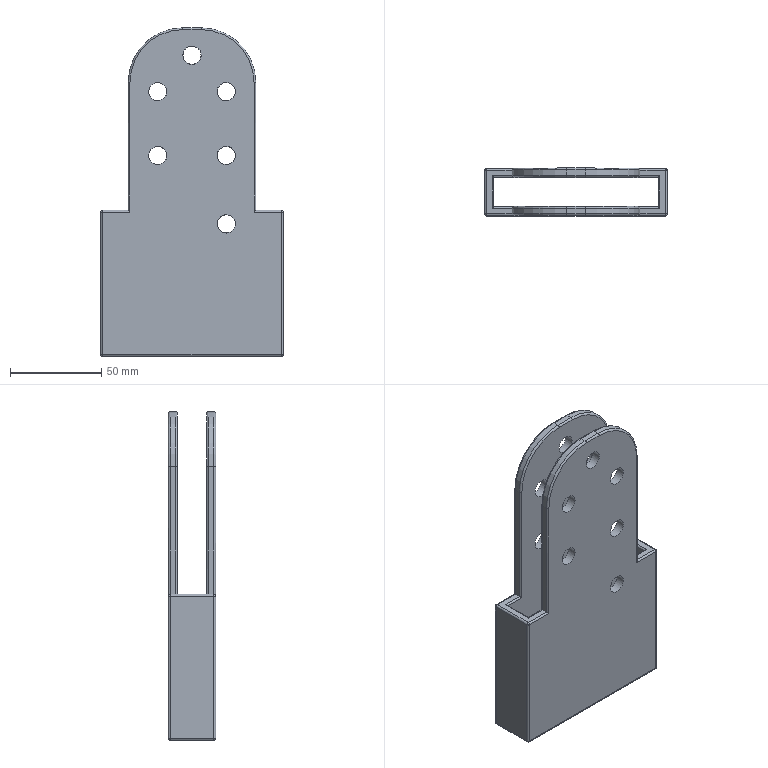Component | NX | JJZ-001 | 1 solid | 91 faces | volume 152795 mm3 | cylinder 57 | plane 18 | torus 8 | sphere 8 | commonest cylinder face diameters 2 x36 10 x14 60 x4 6 x3